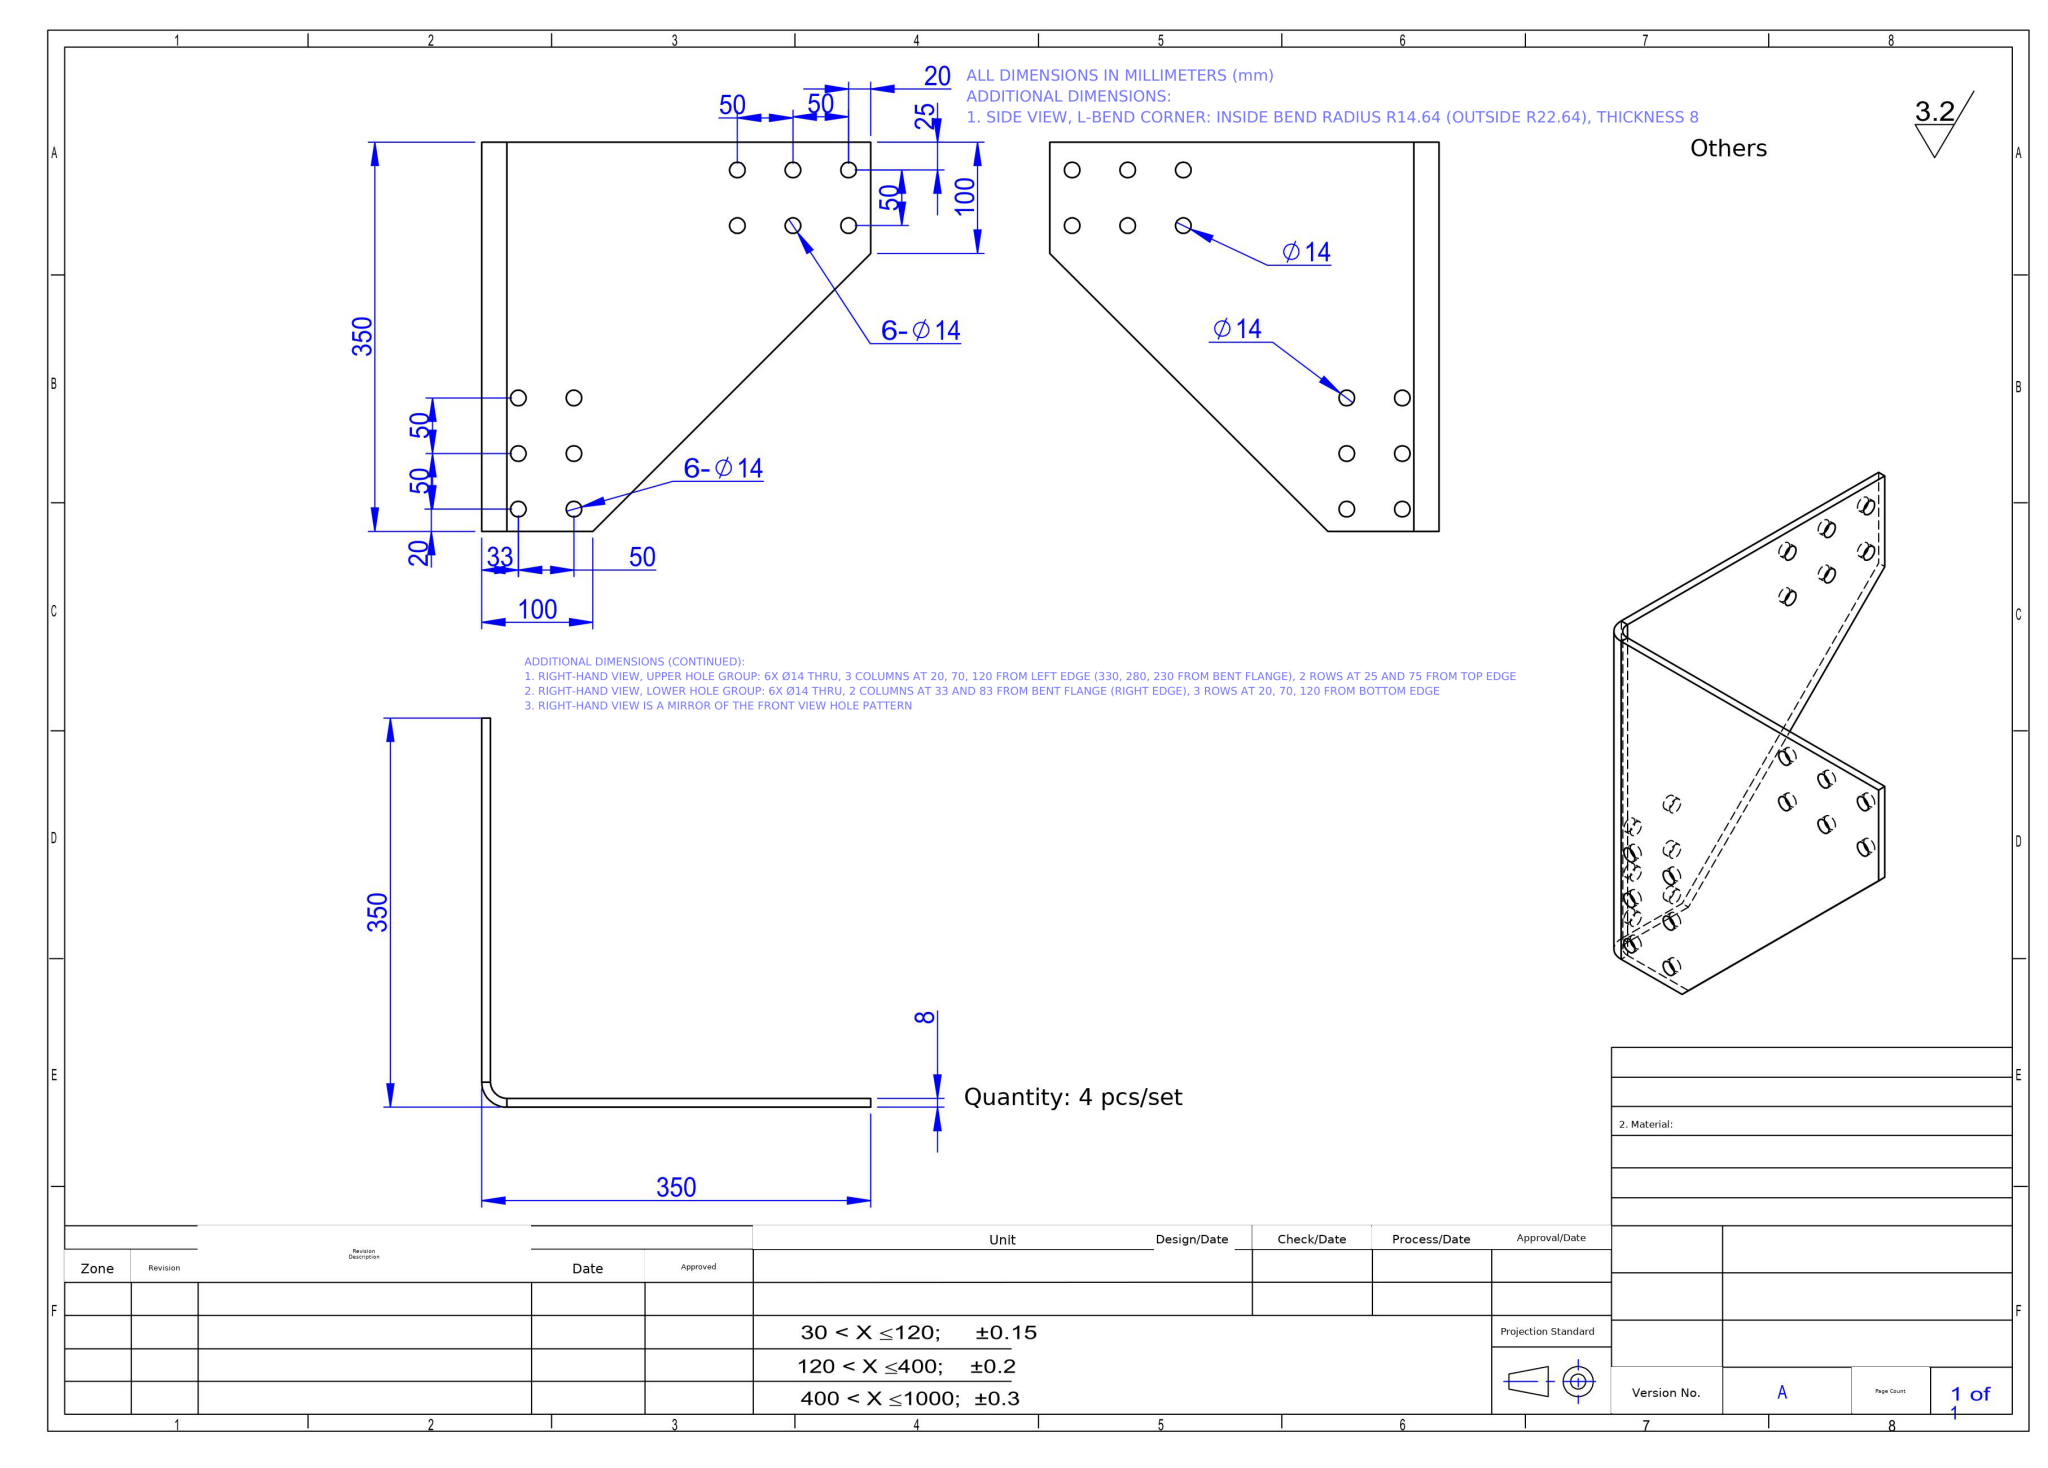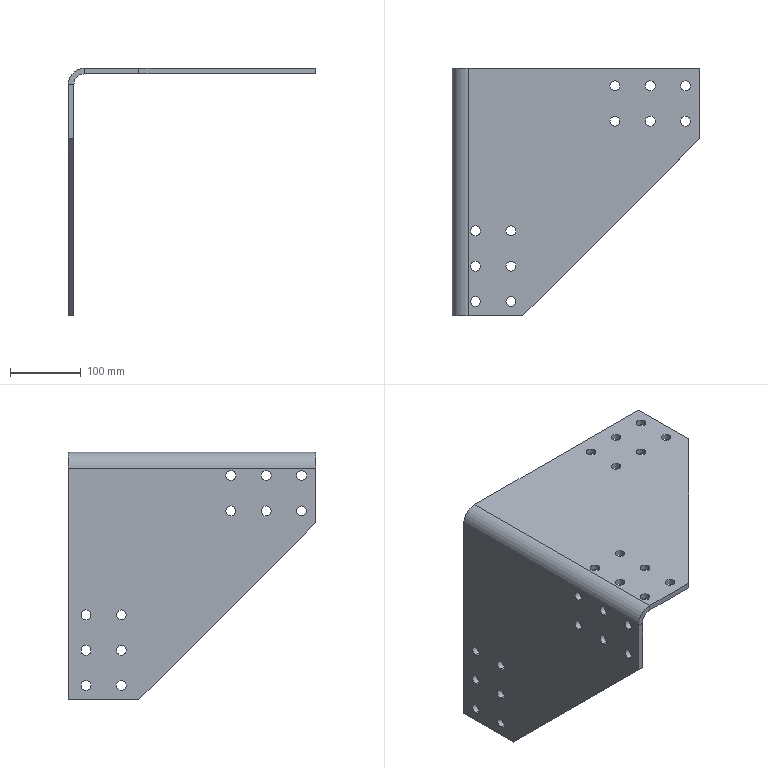Part | NX | mm | 1 solid | 64 faces | box 350 x 350 x 350 mm | volume 1385643 mm3 | cylinder 50 | plane 14 | commonest cylinder face diameters 14 x48 45.28 x1 29.28 x1